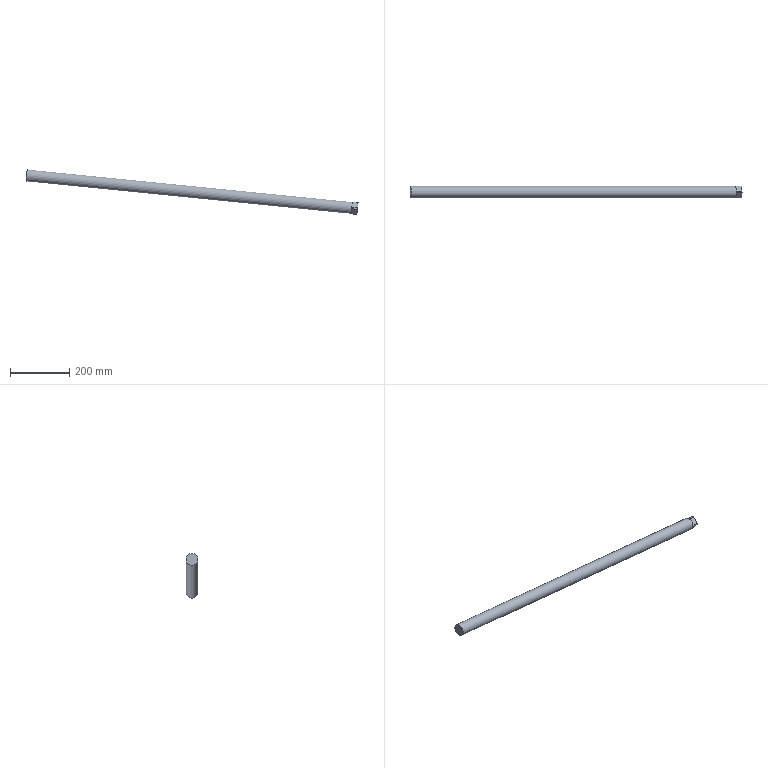Component | NX | ADJUSTTABLE_AXLE1 | 2 solids | 13 faces | box 1123.41 x 40 x 151.52 mm | volume 1408479 mm3 | plane 8 | other 4 | cylinder 1 | commonest cylinder face diameters 40 x1
STEP:
#1=CARTESIAN_POINT('',(0.,0.,0.));
#2=DIRECTION('',(0.,0.,1.));
#3=DIRECTION('',(1.,0.,0.));
#4=AXIS2_PLACEMENT_3D('',#1,#2,#3);
#5=CARTESIAN_POINT('',(1583.185,87.5,396.935));
#6=VERTEX_POINT('',#5);
#7=CARTESIAN_POINT('',(1583.185,67.5,396.935));
#8=DIRECTION('',(0.9951,0.,-0.09932));
#9=DIRECTION('',(0.,1.,0.));
#10=AXIS2_PLACEMENT_3D('',#7,#8,#9);
#11=CIRCLE('',#10,20.);
#12=CARTESIAN_POINT('',(1583.185,67.5,396.935));
#13=DIRECTION('',(-0.9951,0.,0.09932));
#14=DIRECTION('',(0.09932,0.,0.9951));
#15=AXIS2_PLACEMENT_3D('',#12,#13,#14);
#16=CYLINDRICAL_SURFACE('',#15,20.);
#17=CARTESIAN_POINT('',(7.854,0.));
#18=DIRECTION('',(-1.,0.));
#19=VECTOR('',#18,1.);
#20=LINE('',#17,#19);
#21=(GEOMETRIC_REPRESENTATION_CONTEXT(2)PARAMETRIC_REPRESENTATION_CONTEXT()REPRESENTATION_CONTEXT('',''));
#22=DEFINITIONAL_REPRESENTATION('',(#20),#21);
#23=PCURVE('',#16,#22);
#24=CARTESIAN_POINT('',(1583.185,67.5,396.935));
#25=DIRECTION('',(0.9951,0.,-0.09932));
#26=DIRECTION('',(-0.09932,0.,-0.9951));
#27=AXIS2_PLACEMENT_3D('',#24,#25,#26);
#28=PLANE('',#27);
#29=CARTESIAN_POINT('',(0.,0.));
#30=DIRECTION('',(0.,1.));
#31=AXIS2_PLACEMENT_2D('',#29,#30);
#32=CIRCLE('',#31,20.);
#33=(GEOMETRIC_REPRESENTATION_CONTEXT(2)PARAMETRIC_REPRESENTATION_CONTEXT()REPRESENTATION_CONTEXT('',''));
#34=DEFINITIONAL_REPRESENTATION('',(#32),#33);
#35=PCURVE('',#28,#34);
#36=SURFACE_CURVE('',#11,(#23,#35),.PCURVE_S1.);
#37=EDGE_CURVE('',#6,#6,#36,.T.);
#38=ORIENTED_EDGE('',*,*,#37,.F.);
#39=CARTESIAN_POINT('',(483.649,87.5,506.684));
#40=VERTEX_POINT('',#39);
#41=CARTESIAN_POINT('',(1583.185,87.5,396.935));
#42=CARTESIAN_POINT('',(483.649,87.5,506.684));
#43=B_SPLINE_CURVE_WITH_KNOTS('',1,(#41,#42),.UNSPECIFIED.,.F.,.F.,(2,2),(0.,1105.),.PIECEWISE_BEZIER_KNOTS.);
#44=CARTESIAN_POINT('',(7.854,0.));
#45=DIRECTION('',(0.,1.));
#46=VECTOR('',#45,1.);
#47=LINE('',#44,#46);
#48=(GEOMETRIC_REPRESENTATION_CONTEXT(2)PARAMETRIC_REPRESENTATION_CONTEXT()REPRESENTATION_CONTEXT('',''));
#49=DEFINITIONAL_REPRESENTATION('',(#47),#48);
#50=PCURVE('',#16,#49);
#51=CARTESIAN_POINT('',(1.571,0.));
#52=DIRECTION('',(0.,1.));
#53=VECTOR('',#52,1.);
#54=LINE('',#51,#53);
#55=(GEOMETRIC_REPRESENTATION_CONTEXT(2)PARAMETRIC_REPRESENTATION_CONTEXT()REPRESENTATION_CONTEXT('',''));
#56=DEFINITIONAL_REPRESENTATION('',(#54),#55);
#57=PCURVE('',#16,#56);
#58=SEAM_CURVE('',#43,(#50,#57),.PCURVE_S1.);
#59=EDGE_CURVE('',#6,#40,#58,.T.);
#60=ORIENTED_EDGE('',*,*,#59,.T.);
#61=CARTESIAN_POINT('',(483.649,67.5,506.684));
#62=DIRECTION('',(0.9951,0.,-0.09932));
#63=DIRECTION('',(0.,1.,0.));
#64=AXIS2_PLACEMENT_3D('',#61,#62,#63);
#65=CIRCLE('',#64,20.);
#66=CARTESIAN_POINT('',(7.854,1105.));
#67=DIRECTION('',(-1.,0.));
#68=VECTOR('',#67,1.);
#69=LINE('',#66,#68);
#70=(GEOMETRIC_REPRESENTATION_CONTEXT(2)PARAMETRIC_REPRESENTATION_CONTEXT()REPRESENTATION_CONTEXT('',''));
#71=DEFINITIONAL_REPRESENTATION('',(#69),#70);
#72=PCURVE('',#16,#71);
#73=CARTESIAN_POINT('',(483.649,67.5,506.684));
#74=DIRECTION('',(0.9951,0.,-0.09932));
#75=DIRECTION('',(-0.09932,0.,-0.9951));
#76=AXIS2_PLACEMENT_3D('',#73,#74,#75);
#77=PLANE('',#76);
#78=CARTESIAN_POINT('',(0.,0.));
#79=DIRECTION('',(0.,1.));
#80=AXIS2_PLACEMENT_2D('',#78,#79);
#81=CIRCLE('',#80,20.);
#82=(GEOMETRIC_REPRESENTATION_CONTEXT(2)PARAMETRIC_REPRESENTATION_CONTEXT()REPRESENTATION_CONTEXT('',''));
#83=DEFINITIONAL_REPRESENTATION('',(#81),#82);
#84=PCURVE('',#77,#83);
#85=SURFACE_CURVE('',#65,(#72,#84),.PCURVE_S1.);
#86=EDGE_CURVE('',#40,#40,#85,.T.);
#87=ORIENTED_EDGE('',*,*,#86,.T.);
#88=ORIENTED_EDGE('',*,*,#59,.F.);
#89=EDGE_LOOP('',(#38,#60,#87,#88));
#90=FACE_BOUND('',#89,.T.);
#91=ADVANCED_FACE('',(#90),#16,.T.);
#92=ORIENTED_EDGE('',*,*,#37,.T.);
#93=EDGE_LOOP('',(#92));
#94=FACE_BOUND('',#93,.T.);
#95=ADVANCED_FACE('',(#94),#28,.T.);
#96=ORIENTED_EDGE('',*,*,#86,.F.);
#97=EDGE_LOOP('',(#96));
#98=FACE_BOUND('',#97,.T.);
#99=ADVANCED_FACE('',(#98),#77,.F.);
#100=CLOSED_SHELL('',(#91,#95,#99));
#101=MANIFOLD_SOLID_BREP('',#100);
#102=(LENGTH_UNIT()NAMED_UNIT(*)SI_UNIT(.MILLI.,.METRE.));
#103=UNCERTAINTY_MEASURE_WITH_UNIT(LENGTH_MEASURE(0.00001),#102,'','');
#104=(NAMED_UNIT(*)PLANE_ANGLE_UNIT()SI_UNIT($,.RADIAN.));
#105=(NAMED_UNIT(*)SI_UNIT($,.STERADIAN.)SOLID_ANGLE_UNIT());
#106=(GEOMETRIC_REPRESENTATION_CONTEXT(3)GLOBAL_UNCERTAINTY_ASSIGNED_CONTEXT((#103))GLOBAL_UNIT_ASSIGNED_CONTEXT((#102,#104,#105))REPRESENTATION_CONTEXT('',''));
#107=ADVANCED_BREP_SHAPE_REPRESENTATION('',(#4,#101),#106);
#108=CARTESIAN_POINT('',(0.,0.,0.));
#109=DIRECTION('',(0.,0.,1.));
#110=DIRECTION('',(1.,0.,0.));
#111=AXIS2_PLACEMENT_3D('',#108,#109,#110);
#112=CARTESIAN_POINT('',(0.,0.,0.));
#113=DIRECTION('',(0.,0.,1.));
#114=DIRECTION('',(1.,0.,0.));
#115=AXIS2_PLACEMENT_3D('',#112,#113,#114);
#116=(LENGTH_UNIT()NAMED_UNIT(*)SI_UNIT(.MILLI.,.METRE.));
#117=UNCERTAINTY_MEASURE_WITH_UNIT(LENGTH_MEASURE(0.000001),#116,'','');
#118=(NAMED_UNIT(*)PLANE_ANGLE_UNIT()SI_UNIT($,.RADIAN.));
#119=(NAMED_UNIT(*)SI_UNIT($,.STERADIAN.)SOLID_ANGLE_UNIT());
#120=(GEOMETRIC_REPRESENTATION_CONTEXT(3)GLOBAL_UNCERTAINTY_ASSIGNED_CONTEXT((#117))GLOBAL_UNIT_ASSIGNED_CONTEXT((#116,#118,#119))REPRESENTATION_CONTEXT('',''));
#121=SHAPE_REPRESENTATION('',(#4,#111,#115),#120);
#122=ITEM_DEFINED_TRANSFORMATION('','',#4,#111);
#123=(REPRESENTATION_RELATIONSHIP('','',#107,#121)REPRESENTATION_RELATIONSHIP_WITH_TRANSFORMATION(#122)SHAPE_REPRESENTATION_RELATIONSHIP());
#124=CARTESIAN_POINT('',(1603.368,47.704,397.767));
#125=VERTEX_POINT('',#124);
#126=CARTESIAN_POINT('',(1583.467,47.704,399.753));
#127=VERTEX_POINT('',#126);
#128=CARTESIAN_POINT('',(1603.368,47.704,397.767));
#129=DIRECTION('',(-0.9951,0.,0.09932));
#130=VECTOR('',#129,1.);
#131=LINE('',#128,#130);
#132=CARTESIAN_POINT('',(1603.086,67.5,394.949));
#133=DIRECTION('',(0.9951,0.,-0.09932));
#134=DIRECTION('',(0.,1.,0.));
#135=AXIS2_PLACEMENT_3D('',#132,#133,#134);
#136=ELLIPSE('',#135,19.997,19.98);
#137=DIRECTION('',(-0.9951,0.,0.09932));
#138=VECTOR('',#137,1.);
#139=SURFACE_OF_LINEAR_EXTRUSION('',#136,#138);
#140=CARTESIAN_POINT('',(2.999,-0.));
#141=DIRECTION('',(0.,1.));
#142=VECTOR('',#141,1.);
#143=LINE('',#140,#142);
#144=(GEOMETRIC_REPRESENTATION_CONTEXT(2)PARAMETRIC_REPRESENTATION_CONTEXT()REPRESENTATION_CONTEXT('',''));
#145=DEFINITIONAL_REPRESENTATION('',(#143),#144);
#146=PCURVE('',#139,#145);
#147=CARTESIAN_POINT('',(1605.05,64.648,414.627));
#148=DIRECTION('',(-0.07023,0.7071,-0.7036));
#149=DIRECTION('',(0.07023,0.7071,0.7036));
#150=AXIS2_PLACEMENT_3D('',#147,#148,#149);
#151=PLANE('',#150);
#152=CARTESIAN_POINT('',(-23.962,0.));
#153=DIRECTION('',(0.,-1.));
#154=VECTOR('',#153,1.);
#155=LINE('',#152,#154);
#156=(GEOMETRIC_REPRESENTATION_CONTEXT(2)PARAMETRIC_REPRESENTATION_CONTEXT()REPRESENTATION_CONTEXT('',''));
#157=DEFINITIONAL_REPRESENTATION('',(#155),#156);
#158=PCURVE('',#151,#157);
#159=SURFACE_CURVE('',#131,(#146,#158),.PCURVE_S1.);
#160=EDGE_CURVE('',#125,#127,#159,.T.);
#161=ORIENTED_EDGE('',*,*,#160,.F.);
#162=CARTESIAN_POINT('',(1602.805,47.704,392.131));
#163=VERTEX_POINT('',#162);
#164=CARTESIAN_POINT('',(1603.086,67.5,394.949));
#165=DIRECTION('',(0.9951,0.,-0.09932));
#166=DIRECTION('',(0.,1.,0.));
#167=AXIS2_PLACEMENT_3D('',#164,#165,#166);
#168=ELLIPSE('',#167,19.997,19.98);
#169=CARTESIAN_POINT('',(0.,0.));
#170=DIRECTION('',(1.,0.));
#171=VECTOR('',#170,1.);
#172=LINE('',#169,#171);
#173=(GEOMETRIC_REPRESENTATION_CONTEXT(2)PARAMETRIC_REPRESENTATION_CONTEXT()REPRESENTATION_CONTEXT('',''));
#174=DEFINITIONAL_REPRESENTATION('',(#172),#173);
#175=PCURVE('',#139,#174);
#176=CARTESIAN_POINT('',(1603.086,67.5,394.949));
#177=DIRECTION('',(0.9951,0.,-0.09932));
#178=DIRECTION('',(-0.09932,0.,-0.9951));
#179=AXIS2_PLACEMENT_3D('',#176,#177,#178);
#180=PLANE('',#179);
#181=CARTESIAN_POINT('',(0.,0.));
#182=DIRECTION('',(0.,1.));
#183=AXIS2_PLACEMENT_2D('',#181,#182);
#184=ELLIPSE('',#183,19.997,19.98);
#185=(GEOMETRIC_REPRESENTATION_CONTEXT(2)PARAMETRIC_REPRESENTATION_CONTEXT()REPRESENTATION_CONTEXT('',''));
#186=DEFINITIONAL_REPRESENTATION('',(#184),#185);
#187=PCURVE('',#180,#186);
#188=SURFACE_CURVE('',#168,(#175,#187),.PCURVE_S1.);
#189=EDGE_CURVE('',#125,#163,#188,.T.);
#190=ORIENTED_EDGE('',*,*,#189,.T.);
#191=CARTESIAN_POINT('',(1582.904,47.704,394.118));
#192=VERTEX_POINT('',#191);
#193=CARTESIAN_POINT('',(1602.805,47.704,392.131));
#194=DIRECTION('',(-0.9951,0.,0.09932));
#195=VECTOR('',#194,1.);
#196=LINE('',#193,#195);
#197=CARTESIAN_POINT('',(3.284,-0.));
#198=DIRECTION('',(0.,1.));
#199=VECTOR('',#198,1.);
#200=LINE('',#197,#199);
#201=(GEOMETRIC_REPRESENTATION_CONTEXT(2)PARAMETRIC_REPRESENTATION_CONTEXT()REPRESENTATION_CONTEXT('',''));
#202=DEFINITIONAL_REPRESENTATION('',(#200),#201);
#203=PCURVE('',#139,#202);
#204=CARTESIAN_POINT('',(1602.805,47.704,392.131));
#205=DIRECTION('',(0.07023,0.7071,0.7036));
#206=DIRECTION('',(0.07023,-0.7071,0.7036));
#207=AXIS2_PLACEMENT_3D('',#204,#205,#206);
#208=PLANE('',#207);
#209=CARTESIAN_POINT('',(-0.,-0.));
#210=DIRECTION('',(0.,-1.));
#211=VECTOR('',#210,1.);
#212=LINE('',#209,#211);
#213=(GEOMETRIC_REPRESENTATION_CONTEXT(2)PARAMETRIC_REPRESENTATION_CONTEXT()REPRESENTATION_CONTEXT('',''));
#214=DEFINITIONAL_REPRESENTATION('',(#212),#213);
#215=PCURVE('',#208,#214);
#216=SURFACE_CURVE('',#196,(#203,#215),.PCURVE_S1.);
#217=EDGE_CURVE('',#163,#192,#216,.T.);
#218=ORIENTED_EDGE('',*,*,#217,.T.);
#219=CARTESIAN_POINT('',(1583.185,67.5,396.935));
#220=DIRECTION('',(0.9951,0.,-0.09932));
#221=DIRECTION('',(0.,1.,0.));
#222=AXIS2_PLACEMENT_3D('',#219,#220,#221);
#223=ELLIPSE('',#222,19.997,19.98);
#224=CARTESIAN_POINT('',(-0.,20.));
#225=DIRECTION('',(1.,-0.));
#226=VECTOR('',#225,1.);
#227=LINE('',#224,#226);
#228=(GEOMETRIC_REPRESENTATION_CONTEXT(2)PARAMETRIC_REPRESENTATION_CONTEXT()REPRESENTATION_CONTEXT('',''));
#229=DEFINITIONAL_REPRESENTATION('',(#227),#228);
#230=PCURVE('',#139,#229);
#231=CARTESIAN_POINT('',(1583.185,67.5,396.935));
#232=DIRECTION('',(0.9951,0.,-0.09932));
#233=DIRECTION('',(-0.09932,0.,-0.9951));
#234=AXIS2_PLACEMENT_3D('',#231,#232,#233);
#235=PLANE('',#234);
#236=CARTESIAN_POINT('',(0.,0.));
#237=DIRECTION('',(0.,1.));
#238=AXIS2_PLACEMENT_2D('',#236,#237);
#239=ELLIPSE('',#238,19.997,19.98);
#240=(GEOMETRIC_REPRESENTATION_CONTEXT(2)PARAMETRIC_REPRESENTATION_CONTEXT()REPRESENTATION_CONTEXT('',''));
#241=DEFINITIONAL_REPRESENTATION('',(#239),#240);
#242=PCURVE('',#235,#241);
#243=SURFACE_CURVE('',#223,(#230,#242),.PCURVE_S1.);
#244=EDGE_CURVE('',#127,#192,#243,.T.);
#245=ORIENTED_EDGE('',*,*,#244,.F.);
#246=EDGE_LOOP('',(#161,#190,#218,#245));
#247=FACE_BOUND('',#246,.F.);
#248=ADVANCED_FACE('',(#247),#139,.F.);
#249=CARTESIAN_POINT('',(1581.221,64.648,377.258));
#250=VERTEX_POINT('',#249);
#251=CARTESIAN_POINT('',(1582.904,47.704,394.118));
#252=DIRECTION('',(-0.07023,0.7071,-0.7036));
#253=VECTOR('',#252,1.);
#254=LINE('',#251,#253);
#255=CARTESIAN_POINT('',(-0.,-20.));
#256=DIRECTION('',(-1.,-0.));
#257=VECTOR('',#256,1.);
#258=LINE('',#255,#257);
#259=(GEOMETRIC_REPRESENTATION_CONTEXT(2)PARAMETRIC_REPRESENTATION_CONTEXT()REPRESENTATION_CONTEXT('',''));
#260=DEFINITIONAL_REPRESENTATION('',(#258),#259);
#261=PCURVE('',#208,#260);
#262=CARTESIAN_POINT('',(2.832,-19.796));
#263=DIRECTION('',(0.7071,0.7071));
#264=VECTOR('',#263,1.);
#265=LINE('',#262,#264);
#266=(GEOMETRIC_REPRESENTATION_CONTEXT(2)PARAMETRIC_REPRESENTATION_CONTEXT()REPRESENTATION_CONTEXT('',''));
#267=DEFINITIONAL_REPRESENTATION('',(#265),#266);
#268=PCURVE('',#235,#267);
#269=SURFACE_CURVE('',#254,(#261,#268),.PCURVE_S1.);
#270=EDGE_CURVE('',#192,#250,#269,.T.);
#271=ORIENTED_EDGE('',*,*,#270,.T.);
#272=CARTESIAN_POINT('',(1601.122,64.648,375.271));
#273=VERTEX_POINT('',#272);
#274=CARTESIAN_POINT('',(1601.122,64.648,375.271));
#275=DIRECTION('',(-0.9951,0.,0.09932));
#276=VECTOR('',#275,1.);
#277=LINE('',#274,#276);
#278=CARTESIAN_POINT('',(-23.962,-0.));
#279=DIRECTION('',(0.,-1.));
#280=VECTOR('',#279,1.);
#281=LINE('',#278,#280);
#282=(GEOMETRIC_REPRESENTATION_CONTEXT(2)PARAMETRIC_REPRESENTATION_CONTEXT()REPRESENTATION_CONTEXT('',''));
#283=DEFINITIONAL_REPRESENTATION('',(#281),#282);
#284=PCURVE('',#208,#283);
#285=CARTESIAN_POINT('',(1603.086,67.5,394.949));
#286=DIRECTION('',(0.9951,0.,-0.09932));
#287=DIRECTION('',(0.,1.,0.));
#288=AXIS2_PLACEMENT_3D('',#285,#286,#287);
#289=ELLIPSE('',#288,19.997,19.98);
#290=DIRECTION('',(-0.9951,0.,0.09932));
#291=VECTOR('',#290,1.);
#292=SURFACE_OF_LINEAR_EXTRUSION('',#289,#291);
#293=CARTESIAN_POINT('',(4.569,-0.));
#294=DIRECTION('',(0.,1.));
#295=VECTOR('',#294,1.);
#296=LINE('',#293,#295);
#297=(GEOMETRIC_REPRESENTATION_CONTEXT(2)PARAMETRIC_REPRESENTATION_CONTEXT()REPRESENTATION_CONTEXT('',''));
#298=DEFINITIONAL_REPRESENTATION('',(#296),#297);
#299=PCURVE('',#292,#298);
#300=SURFACE_CURVE('',#277,(#284,#299),.PCURVE_S1.);
#301=EDGE_CURVE('',#273,#250,#300,.T.);
#302=ORIENTED_EDGE('',*,*,#301,.F.);
#303=CARTESIAN_POINT('',(1602.805,47.704,392.131));
#304=DIRECTION('',(-0.07023,0.7071,-0.7036));
#305=VECTOR('',#304,1.);
#306=LINE('',#303,#305);
#307=CARTESIAN_POINT('',(0.,0.));
#308=DIRECTION('',(-1.,-0.));
#309=VECTOR('',#308,1.);
#310=LINE('',#307,#309);
#311=(GEOMETRIC_REPRESENTATION_CONTEXT(2)PARAMETRIC_REPRESENTATION_CONTEXT()REPRESENTATION_CONTEXT('',''));
#312=DEFINITIONAL_REPRESENTATION('',(#310),#311);
#313=PCURVE('',#208,#312);
#314=CARTESIAN_POINT('',(2.832,-19.796));
#315=DIRECTION('',(0.7071,0.7071));
#316=VECTOR('',#315,1.);
#317=LINE('',#314,#316);
#318=(GEOMETRIC_REPRESENTATION_CONTEXT(2)PARAMETRIC_REPRESENTATION_CONTEXT()REPRESENTATION_CONTEXT('',''));
#319=DEFINITIONAL_REPRESENTATION('',(#317),#318);
#320=PCURVE('',#180,#319);
#321=SURFACE_CURVE('',#306,(#313,#320),.PCURVE_S1.);
#322=EDGE_CURVE('',#163,#273,#321,.T.);
#323=ORIENTED_EDGE('',*,*,#322,.F.);
#324=ORIENTED_EDGE('',*,*,#217,.T.);
#325=EDGE_LOOP('',(#271,#302,#323,#324));
#326=FACE_BOUND('',#325,.T.);
#327=ADVANCED_FACE('',(#326),#208,.F.);
#328=ORIENTED_EDGE('',*,*,#301,.F.);
#329=CARTESIAN_POINT('',(1601.122,70.352,375.271));
#330=VERTEX_POINT('',#329);
#331=CARTESIAN_POINT('',(1603.086,67.5,394.949));
#332=DIRECTION('',(0.9951,0.,-0.09932));
#333=DIRECTION('',(0.,1.,0.));
#334=AXIS2_PLACEMENT_3D('',#331,#332,#333);
#335=ELLIPSE('',#334,19.997,19.98);
#336=CARTESIAN_POINT('',(0.,0.));
#337=DIRECTION('',(1.,0.));
#338=VECTOR('',#337,1.);
#339=LINE('',#336,#338);
#340=(GEOMETRIC_REPRESENTATION_CONTEXT(2)PARAMETRIC_REPRESENTATION_CONTEXT()REPRESENTATION_CONTEXT('',''));
#341=DEFINITIONAL_REPRESENTATION('',(#339),#340);
#342=PCURVE('',#292,#341);
#343=CARTESIAN_POINT('',(0.,0.));
#344=DIRECTION('',(0.,1.));
#345=AXIS2_PLACEMENT_2D('',#343,#344);
#346=ELLIPSE('',#345,19.997,19.98);
#347=(GEOMETRIC_REPRESENTATION_CONTEXT(2)PARAMETRIC_REPRESENTATION_CONTEXT()REPRESENTATION_CONTEXT('',''));
#348=DEFINITIONAL_REPRESENTATION('',(#346),#347);
#349=PCURVE('',#180,#348);
#350=SURFACE_CURVE('',#335,(#342,#349),.PCURVE_S1.);
#351=EDGE_CURVE('',#273,#330,#350,.T.);
#352=ORIENTED_EDGE('',*,*,#351,.T.);
#353=CARTESIAN_POINT('',(1581.221,70.352,377.258));
#354=VERTEX_POINT('',#353);
#355=CARTESIAN_POINT('',(1601.122,70.352,375.271));
#356=DIRECTION('',(-0.9951,0.,0.09932));
#357=VECTOR('',#356,1.);
#358=LINE('',#355,#357);
#359=CARTESIAN_POINT('',(4.855,-0.));
#360=DIRECTION('',(-0.,1.));
#361=VECTOR('',#360,1.);
#362=LINE('',#359,#361);
#363=(GEOMETRIC_REPRESENTATION_CONTEXT(2)PARAMETRIC_REPRESENTATION_CONTEXT()REPRESENTATION_CONTEXT('',''));
#364=DEFINITIONAL_REPRESENTATION('',(#362),#363);
#365=PCURVE('',#292,#364);
#366=CARTESIAN_POINT('',(1601.122,70.352,375.271));
#367=DIRECTION('',(0.07023,-0.7071,0.7036));
#368=DIRECTION('',(-0.07023,-0.7071,-0.7036));
#369=AXIS2_PLACEMENT_3D('',#366,#367,#368);
#370=PLANE('',#369);
#371=CARTESIAN_POINT('',(0.,0.));
#372=DIRECTION('',(0.,-1.));
#373=VECTOR('',#372,1.);
#374=LINE('',#371,#373);
#375=(GEOMETRIC_REPRESENTATION_CONTEXT(2)PARAMETRIC_REPRESENTATION_CONTEXT()REPRESENTATION_CONTEXT('',''));
#376=DEFINITIONAL_REPRESENTATION('',(#374),#375);
#377=PCURVE('',#370,#376);
#378=SURFACE_CURVE('',#358,(#365,#377),.PCURVE_S1.);
#379=EDGE_CURVE('',#330,#354,#378,.T.);
#380=ORIENTED_EDGE('',*,*,#379,.T.);
#381=CARTESIAN_POINT('',(1583.185,67.5,396.935));
#382=DIRECTION('',(0.9951,0.,-0.09932));
#383=DIRECTION('',(0.,1.,0.));
#384=AXIS2_PLACEMENT_3D('',#381,#382,#383);
#385=ELLIPSE('',#384,19.997,19.98);
#386=CARTESIAN_POINT('',(-0.,20.));
#387=DIRECTION('',(1.,0.));
#388=VECTOR('',#387,1.);
#389=LINE('',#386,#388);
#390=(GEOMETRIC_REPRESENTATION_CONTEXT(2)PARAMETRIC_REPRESENTATION_CONTEXT()REPRESENTATION_CONTEXT('',''));
#391=DEFINITIONAL_REPRESENTATION('',(#389),#390);
#392=PCURVE('',#292,#391);
#393=CARTESIAN_POINT('',(0.,0.));
#394=DIRECTION('',(0.,1.));
#395=AXIS2_PLACEMENT_2D('',#393,#394);
#396=ELLIPSE('',#395,19.997,19.98);
#397=(GEOMETRIC_REPRESENTATION_CONTEXT(2)PARAMETRIC_REPRESENTATION_CONTEXT()REPRESENTATION_CONTEXT('',''));
#398=DEFINITIONAL_REPRESENTATION('',(#396),#397);
#399=PCURVE('',#235,#398);
#400=SURFACE_CURVE('',#385,(#392,#399),.PCURVE_S1.);
#401=EDGE_CURVE('',#250,#354,#400,.T.);
#402=ORIENTED_EDGE('',*,*,#401,.F.);
#403=EDGE_LOOP('',(#328,#352,#380,#402));
#404=FACE_BOUND('',#403,.F.);
#405=ADVANCED_FACE('',(#404),#292,.F.);
#406=CARTESIAN_POINT('',(1582.904,87.296,394.118));
#407=VERTEX_POINT('',#406);
#408=CARTESIAN_POINT('',(1581.221,70.352,377.258));
#409=DIRECTION('',(0.07023,0.7071,0.7036));
#410=VECTOR('',#409,1.);
#411=LINE('',#408,#410);
#412=CARTESIAN_POINT('',(-0.,-20.));
#413=DIRECTION('',(-1.,-0.));
#414=VECTOR('',#413,1.);
#415=LINE('',#412,#414);
#416=(GEOMETRIC_REPRESENTATION_CONTEXT(2)PARAMETRIC_REPRESENTATION_CONTEXT()REPRESENTATION_CONTEXT('',''));
#417=DEFINITIONAL_REPRESENTATION('',(#415),#416);
#418=PCURVE('',#370,#417);
#419=CARTESIAN_POINT('',(19.775,2.852));
#420=DIRECTION('',(-0.7071,0.7071));
#421=VECTOR('',#420,1.);
#422=LINE('',#419,#421);
#423=(GEOMETRIC_REPRESENTATION_CONTEXT(2)PARAMETRIC_REPRESENTATION_CONTEXT()REPRESENTATION_CONTEXT('',''));
#424=DEFINITIONAL_REPRESENTATION('',(#422),#423);
#425=PCURVE('',#235,#424);
#426=SURFACE_CURVE('',#411,(#418,#425),.PCURVE_S1.);
#427=EDGE_CURVE('',#354,#407,#426,.T.);
#428=ORIENTED_EDGE('',*,*,#427,.T.);
#429=CARTESIAN_POINT('',(1602.805,87.296,392.131));
#430=VERTEX_POINT('',#429);
#431=CARTESIAN_POINT('',(1602.805,87.296,392.131));
#432=DIRECTION('',(-0.9951,0.,0.09932));
#433=VECTOR('',#432,1.);
#434=LINE('',#431,#433);
#435=CARTESIAN_POINT('',(-23.962,0.));
#436=DIRECTION('',(0.,-1.));
#437=VECTOR('',#436,1.);
#438=LINE('',#435,#437);
#439=(GEOMETRIC_REPRESENTATION_CONTEXT(2)PARAMETRIC_REPRESENTATION_CONTEXT()REPRESENTATION_CONTEXT('',''));
#440=DEFINITIONAL_REPRESENTATION('',(#438),#439);
#441=PCURVE('',#370,#440);
#442=CARTESIAN_POINT('',(1603.086,67.5,394.949));
#443=DIRECTION('',(0.9951,0.,-0.09932));
#444=DIRECTION('',(0.,1.,0.));
#445=AXIS2_PLACEMENT_3D('',#442,#443,#444);
#446=ELLIPSE('',#445,19.997,19.98);
#447=DIRECTION('',(-0.9951,0.,0.09932));
#448=VECTOR('',#447,1.);
#449=SURFACE_OF_LINEAR_EXTRUSION('',#446,#448);
#450=CARTESIAN_POINT('',(-0.1422,-0.));
#451=DIRECTION('',(0.,1.));
#452=VECTOR('',#451,1.);
#453=LINE('',#450,#452);
#454=(GEOMETRIC_REPRESENTATION_CONTEXT(2)PARAMETRIC_REPRESENTATION_CONTEXT()REPRESENTATION_CONTEXT('',''));
#455=DEFINITIONAL_REPRESENTATION('',(#453),#454);
#456=PCURVE('',#449,#455);
#457=SURFACE_CURVE('',#434,(#441,#456),.PCURVE_S1.);
#458=EDGE_CURVE('',#430,#407,#457,.T.);
#459=ORIENTED_EDGE('',*,*,#458,.F.);
#460=CARTESIAN_POINT('',(1601.122,70.352,375.271));
#461=DIRECTION('',(0.07023,0.7071,0.7036));
#462=VECTOR('',#461,1.);
#463=LINE('',#460,#462);
#464=CARTESIAN_POINT('',(0.,0.));
#465=DIRECTION('',(-1.,-0.));
#466=VECTOR('',#465,1.);
#467=LINE('',#464,#466);
#468=(GEOMETRIC_REPRESENTATION_CONTEXT(2)PARAMETRIC_REPRESENTATION_CONTEXT()REPRESENTATION_CONTEXT('',''));
#469=DEFINITIONAL_REPRESENTATION('',(#467),#468);
#470=PCURVE('',#370,#469);
#471=CARTESIAN_POINT('',(19.775,2.852));
#472=DIRECTION('',(-0.7071,0.7071));
#473=VECTOR('',#472,1.);
#474=LINE('',#471,#473);
#475=(GEOMETRIC_REPRESENTATION_CONTEXT(2)PARAMETRIC_REPRESENTATION_CONTEXT()REPRESENTATION_CONTEXT('',''));
#476=DEFINITIONAL_REPRESENTATION('',(#474),#475);
#477=PCURVE('',#180,#476);
#478=SURFACE_CURVE('',#463,(#470,#477),.PCURVE_S1.);
#479=EDGE_CURVE('',#330,#430,#478,.T.);
#480=ORIENTED_EDGE('',*,*,#479,.F.);
#481=ORIENTED_EDGE('',*,*,#379,.T.);
#482=EDGE_LOOP('',(#428,#459,#480,#481));
#483=FACE_BOUND('',#482,.T.);
#484=ADVANCED_FACE('',(#483),#370,.F.);
#485=ORIENTED_EDGE('',*,*,#458,.F.);
#486=CARTESIAN_POINT('',(1603.368,87.296,397.767));
#487=VERTEX_POINT('',#486);
#488=CARTESIAN_POINT('',(1603.086,67.5,394.949));
#489=DIRECTION('',(0.9951,0.,-0.09932));
#490=DIRECTION('',(0.,1.,0.));
#491=AXIS2_PLACEMENT_3D('',#488,#489,#490);
#492=ELLIPSE('',#491,19.997,19.98);
#493=CARTESIAN_POINT('',(-6.283,-0.));
#494=DIRECTION('',(1.,0.));
#495=VECTOR('',#494,1.);
#496=LINE('',#493,#495);
#497=(GEOMETRIC_REPRESENTATION_CONTEXT(2)PARAMETRIC_REPRESENTATION_CONTEXT()REPRESENTATION_CONTEXT('',''));
#498=DEFINITIONAL_REPRESENTATION('',(#496),#497);
#499=PCURVE('',#449,#498);
#500=CARTESIAN_POINT('',(0.,0.));
#501=DIRECTION('',(0.,1.));
#502=AXIS2_PLACEMENT_2D('',#500,#501);
#503=ELLIPSE('',#502,19.997,19.98);
#504=(GEOMETRIC_REPRESENTATION_CONTEXT(2)PARAMETRIC_REPRESENTATION_CONTEXT()REPRESENTATION_CONTEXT('',''));
#505=DEFINITIONAL_REPRESENTATION('',(#503),#504);
#506=PCURVE('',#180,#505);
#507=SURFACE_CURVE('',#492,(#499,#506),.PCURVE_S1.);
#508=EDGE_CURVE('',#430,#487,#507,.T.);
#509=ORIENTED_EDGE('',*,*,#508,.T.);
#510=CARTESIAN_POINT('',(1583.467,87.296,399.753));
#511=VERTEX_POINT('',#510);
#512=CARTESIAN_POINT('',(1603.368,87.296,397.767));
#513=DIRECTION('',(-0.9951,0.,0.09932));
#514=VECTOR('',#513,1.);
#515=LINE('',#512,#514);
#516=CARTESIAN_POINT('',(0.1422,-0.));
#517=DIRECTION('',(0.,1.));
#518=VECTOR('',#517,1.);
#519=LINE('',#516,#518);
#520=(GEOMETRIC_REPRESENTATION_CONTEXT(2)PARAMETRIC_REPRESENTATION_CONTEXT()REPRESENTATION_CONTEXT('',''));
#521=DEFINITIONAL_REPRESENTATION('',(#519),#520);
#522=PCURVE('',#449,#521);
#523=CARTESIAN_POINT('',(1603.368,87.296,397.767));
#524=DIRECTION('',(-0.07023,-0.7071,-0.7036));
#525=DIRECTION('',(-0.07023,0.7071,-0.7036));
#526=AXIS2_PLACEMENT_3D('',#523,#524,#525);
#527=PLANE('',#526);
#528=CARTESIAN_POINT('',(0.,0.));
#529=DIRECTION('',(0.,-1.));
#530=VECTOR('',#529,1.);
#531=LINE('',#528,#530);
#532=(GEOMETRIC_REPRESENTATION_CONTEXT(2)PARAMETRIC_REPRESENTATION_CONTEXT()REPRESENTATION_CONTEXT('',''));
#533=DEFINITIONAL_REPRESENTATION('',(#531),#532);
#534=PCURVE('',#527,#533);
#535=SURFACE_CURVE('',#515,(#522,#534),.PCURVE_S1.);
#536=EDGE_CURVE('',#487,#511,#535,.T.);
#537=ORIENTED_EDGE('',*,*,#536,.T.);
#538=CARTESIAN_POINT('',(1583.185,67.5,396.935));
#539=DIRECTION('',(0.9951,0.,-0.09932));
#540=DIRECTION('',(0.,1.,0.));
#541=AXIS2_PLACEMENT_3D('',#538,#539,#540);
#542=ELLIPSE('',#541,19.997,19.98);
#543=CARTESIAN_POINT('',(-6.283,20.));
#544=DIRECTION('',(1.,0.));
#545=VECTOR('',#544,1.);
#546=LINE('',#543,#545);
#547=(GEOMETRIC_REPRESENTATION_CONTEXT(2)PARAMETRIC_REPRESENTATION_CONTEXT()REPRESENTATION_CONTEXT('',''));
#548=DEFINITIONAL_REPRESENTATION('',(#546),#547);
#549=PCURVE('',#449,#548);
#550=CARTESIAN_POINT('',(0.,0.));
#551=DIRECTION('',(0.,1.));
#552=AXIS2_PLACEMENT_2D('',#550,#551);
#553=ELLIPSE('',#552,19.997,19.98);
#554=(GEOMETRIC_REPRESENTATION_CONTEXT(2)PARAMETRIC_REPRESENTATION_CONTEXT()REPRESENTATION_CONTEXT('',''));
#555=DEFINITIONAL_REPRESENTATION('',(#553),#554);
#556=PCURVE('',#235,#555);
#557=SURFACE_CURVE('',#542,(#549,#556),.PCURVE_S1.);
#558=EDGE_CURVE('',#407,#511,#557,.T.);
#559=ORIENTED_EDGE('',*,*,#558,.F.);
#560=EDGE_LOOP('',(#485,#509,#537,#559));
#561=FACE_BOUND('',#560,.F.);
#562=ADVANCED_FACE('',(#561),#449,.F.);
#563=CARTESIAN_POINT('',(1585.149,70.352,416.613));
#564=VERTEX_POINT('',#563);
#565=CARTESIAN_POINT('',(1583.467,87.296,399.753));
#566=DIRECTION('',(0.07023,-0.7071,0.7036));
#567=VECTOR('',#566,1.);
#568=LINE('',#565,#567);
#569=CARTESIAN_POINT('',(-0.,-20.));
#570=DIRECTION('',(-1.,-0.));
#571=VECTOR('',#570,1.);
#572=LINE('',#569,#571);
#573=(GEOMETRIC_REPRESENTATION_CONTEXT(2)PARAMETRIC_REPRESENTATION_CONTEXT()REPRESENTATION_CONTEXT('',''));
#574=DEFINITIONAL_REPRESENTATION('',(#572),#573);
#575=PCURVE('',#527,#574);
#576=CARTESIAN_POINT('',(-2.832,19.796));
#577=DIRECTION('',(-0.7071,-0.7071));
#578=VECTOR('',#577,1.);
#579=LINE('',#576,#578);
#580=(GEOMETRIC_REPRESENTATION_CONTEXT(2)PARAMETRIC_REPRESENTATION_CONTEXT()REPRESENTATION_CONTEXT('',''));
#581=DEFINITIONAL_REPRESENTATION('',(#579),#580);
#582=PCURVE('',#235,#581);
#583=SURFACE_CURVE('',#568,(#575,#582),.PCURVE_S1.);
#584=EDGE_CURVE('',#511,#564,#583,.T.);
#585=ORIENTED_EDGE('',*,*,#584,.T.);
#586=CARTESIAN_POINT('',(1605.05,70.352,414.627));
#587=VERTEX_POINT('',#586);
#588=CARTESIAN_POINT('',(1605.05,70.352,414.627));
#589=DIRECTION('',(-0.9951,0.,0.09932));
#590=VECTOR('',#589,1.);
#591=LINE('',#588,#590);
#592=CARTESIAN_POINT('',(-23.962,0.));
#593=DIRECTION('',(0.,-1.));
#594=VECTOR('',#593,1.);
#595=LINE('',#592,#594);
#596=(GEOMETRIC_REPRESENTATION_CONTEXT(2)PARAMETRIC_REPRESENTATION_CONTEXT()REPRESENTATION_CONTEXT('',''));
#597=DEFINITIONAL_REPRESENTATION('',(#595),#596);
#598=PCURVE('',#527,#597);
#599=CARTESIAN_POINT('',(1603.086,67.5,394.949));
#600=DIRECTION('',(0.9951,0.,-0.09932));
#601=DIRECTION('',(0.,1.,0.));
#602=AXIS2_PLACEMENT_3D('',#599,#600,#601);
#603=ELLIPSE('',#602,19.997,19.98);
#604=DIRECTION('',(-0.9951,0.,0.09932));
#605=VECTOR('',#604,1.);
#606=SURFACE_OF_LINEAR_EXTRUSION('',#603,#605);
#607=CARTESIAN_POINT('',(1.428,-0.));
#608=DIRECTION('',(0.,1.));
#609=VECTOR('',#608,1.);
#610=LINE('',#607,#609);
#611=(GEOMETRIC_REPRESENTATION_CONTEXT(2)PARAMETRIC_REPRESENTATION_CONTEXT()REPRESENTATION_CONTEXT('',''));
#612=DEFINITIONAL_REPRESENTATION('',(#610),#611);
#613=PCURVE('',#606,#612);
#614=SURFACE_CURVE('',#591,(#598,#613),.PCURVE_S1.);
#615=EDGE_CURVE('',#587,#564,#614,.T.);
#616=ORIENTED_EDGE('',*,*,#615,.F.);
#617=CARTESIAN_POINT('',(1603.368,87.296,397.767));
#618=DIRECTION('',(0.07023,-0.7071,0.7036));
#619=VECTOR('',#618,1.);
#620=LINE('',#617,#619);
#621=CARTESIAN_POINT('',(0.,0.));
#622=DIRECTION('',(-1.,-0.));
#623=VECTOR('',#622,1.);
#624=LINE('',#621,#623);
#625=(GEOMETRIC_REPRESENTATION_CONTEXT(2)PARAMETRIC_REPRESENTATION_CONTEXT()REPRESENTATION_CONTEXT('',''));
#626=DEFINITIONAL_REPRESENTATION('',(#624),#625);
#627=PCURVE('',#527,#626);
#628=CARTESIAN_POINT('',(-2.832,19.796));
#629=DIRECTION('',(-0.7071,-0.7071));
#630=VECTOR('',#629,1.);
#631=LINE('',#628,#630);
#632=(GEOMETRIC_REPRESENTATION_CONTEXT(2)PARAMETRIC_REPRESENTATION_CONTEXT()REPRESENTATION_CONTEXT('',''));
#633=DEFINITIONAL_REPRESENTATION('',(#631),#632);
#634=PCURVE('',#180,#633);
#635=SURFACE_CURVE('',#620,(#627,#634),.PCURVE_S1.);
#636=EDGE_CURVE('',#487,#587,#635,.T.);
#637=ORIENTED_EDGE('',*,*,#636,.F.);
#638=ORIENTED_EDGE('',*,*,#536,.T.);
#639=EDGE_LOOP('',(#585,#616,#637,#638));
#640=FACE_BOUND('',#639,.T.);
#641=ADVANCED_FACE('',(#640),#527,.F.);
#642=ORIENTED_EDGE('',*,*,#615,.F.);
#643=CARTESIAN_POINT('',(1605.05,64.648,414.627));
#644=VERTEX_POINT('',#643);
#645=CARTESIAN_POINT('',(1603.086,67.5,394.949));
#646=DIRECTION('',(0.9951,0.,-0.09932));
#647=DIRECTION('',(0.,1.,0.));
#648=AXIS2_PLACEMENT_3D('',#645,#646,#647);
#649=ELLIPSE('',#648,19.997,19.98);
#650=CARTESIAN_POINT('',(0.,-0.));
#651=DIRECTION('',(1.,0.));
#652=VECTOR('',#651,1.);
#653=LINE('',#650,#652);
#654=(GEOMETRIC_REPRESENTATION_CONTEXT(2)PARAMETRIC_REPRESENTATION_CONTEXT()REPRESENTATION_CONTEXT('',''));
#655=DEFINITIONAL_REPRESENTATION('',(#653),#654);
#656=PCURVE('',#606,#655);
#657=CARTESIAN_POINT('',(0.,0.));
#658=DIRECTION('',(0.,1.));
#659=AXIS2_PLACEMENT_2D('',#657,#658);
#660=ELLIPSE('',#659,19.997,19.98);
#661=(GEOMETRIC_REPRESENTATION_CONTEXT(2)PARAMETRIC_REPRESENTATION_CONTEXT()REPRESENTATION_CONTEXT('',''));
#662=DEFINITIONAL_REPRESENTATION('',(#660),#661);
#663=PCURVE('',#180,#662);
#664=SURFACE_CURVE('',#649,(#656,#663),.PCURVE_S1.);
#665=EDGE_CURVE('',#587,#644,#664,.T.);
#666=ORIENTED_EDGE('',*,*,#665,.T.);
#667=CARTESIAN_POINT('',(1585.149,64.648,416.613));
#668=VERTEX_POINT('',#667);
#669=CARTESIAN_POINT('',(1605.05,64.648,414.627));
#670=DIRECTION('',(-0.9951,0.,0.09932));
#671=VECTOR('',#670,1.);
#672=LINE('',#669,#671);
#673=CARTESIAN_POINT('',(1.714,-0.));
#674=DIRECTION('',(0.,1.));
#675=VECTOR('',#674,1.);
#676=LINE('',#673,#675);
#677=(GEOMETRIC_REPRESENTATION_CONTEXT(2)PARAMETRIC_REPRESENTATION_CONTEXT()REPRESENTATION_CONTEXT('',''));
#678=DEFINITIONAL_REPRESENTATION('',(#676),#677);
#679=PCURVE('',#606,#678);
#680=CARTESIAN_POINT('',(0.,0.));
#681=DIRECTION('',(0.,-1.));
#682=VECTOR('',#681,1.);
#683=LINE('',#680,#682);
#684=(GEOMETRIC_REPRESENTATION_CONTEXT(2)PARAMETRIC_REPRESENTATION_CONTEXT()REPRESENTATION_CONTEXT('',''));
#685=DEFINITIONAL_REPRESENTATION('',(#683),#684);
#686=PCURVE('',#151,#685);
#687=SURFACE_CURVE('',#672,(#679,#686),.PCURVE_S1.);
#688=EDGE_CURVE('',#644,#668,#687,.T.);
#689=ORIENTED_EDGE('',*,*,#688,.T.);
#690=CARTESIAN_POINT('',(1583.185,67.5,396.935));
#691=DIRECTION('',(0.9951,0.,-0.09932));
#692=DIRECTION('',(0.,1.,0.));
#693=AXIS2_PLACEMENT_3D('',#690,#691,#692);
#694=ELLIPSE('',#693,19.997,19.98);
#695=CARTESIAN_POINT('',(0.,20.));
#696=DIRECTION('',(1.,0.));
#697=VECTOR('',#696,1.);
#698=LINE('',#695,#697);
#699=(GEOMETRIC_REPRESENTATION_CONTEXT(2)PARAMETRIC_REPRESENTATION_CONTEXT()REPRESENTATION_CONTEXT('',''));
#700=DEFINITIONAL_REPRESENTATION('',(#698),#699);
#701=PCURVE('',#606,#700);
#702=CARTESIAN_POINT('',(0.,0.));
#703=DIRECTION('',(0.,1.));
#704=AXIS2_PLACEMENT_2D('',#702,#703);
#705=ELLIPSE('',#704,19.997,19.98);
#706=(GEOMETRIC_REPRESENTATION_CONTEXT(2)PARAMETRIC_REPRESENTATION_CONTEXT()REPRESENTATION_CONTEXT('',''));
#707=DEFINITIONAL_REPRESENTATION('',(#705),#706);
#708=PCURVE('',#235,#707);
#709=SURFACE_CURVE('',#694,(#701,#708),.PCURVE_S1.);
#710=EDGE_CURVE('',#564,#668,#709,.T.);
#711=ORIENTED_EDGE('',*,*,#710,.F.);
#712=EDGE_LOOP('',(#642,#666,#689,#711));
#713=FACE_BOUND('',#712,.F.);
#714=ADVANCED_FACE('',(#713),#606,.F.);
#715=CARTESIAN_POINT('',(1585.149,64.648,416.613));
#716=DIRECTION('',(-0.07023,-0.7071,-0.7036));
#717=VECTOR('',#716,1.);
#718=LINE('',#715,#717);
#719=CARTESIAN_POINT('',(-0.,-20.));
#720=DIRECTION('',(-1.,-0.));
#721=VECTOR('',#720,1.);
#722=LINE('',#719,#721);
#723=(GEOMETRIC_REPRESENTATION_CONTEXT(2)PARAMETRIC_REPRESENTATION_CONTEXT()REPRESENTATION_CONTEXT('',''));
#724=DEFINITIONAL_REPRESENTATION('',(#722),#723);
#725=PCURVE('',#151,#724);
#726=CARTESIAN_POINT('',(-19.775,-2.852));
#727=DIRECTION('',(0.7071,-0.7071));
#728=VECTOR('',#727,1.);
#729=LINE('',#726,#728);
#730=(GEOMETRIC_REPRESENTATION_CONTEXT(2)PARAMETRIC_REPRESENTATION_CONTEXT()REPRESENTATION_CONTEXT('',''));
#731=DEFINITIONAL_REPRESENTATION('',(#729),#730);
#732=PCURVE('',#235,#731);
#733=SURFACE_CURVE('',#718,(#725,#732),.PCURVE_S1.);
#734=EDGE_CURVE('',#668,#127,#733,.T.);
#735=ORIENTED_EDGE('',*,*,#734,.T.);
#736=ORIENTED_EDGE('',*,*,#160,.F.);
#737=CARTESIAN_POINT('',(1605.05,64.648,414.627));
#738=DIRECTION('',(-0.07023,-0.7071,-0.7036));
#739=VECTOR('',#738,1.);
#740=LINE('',#737,#739);
#741=CARTESIAN_POINT('',(0.,0.));
#742=DIRECTION('',(-1.,-0.));
#743=VECTOR('',#742,1.);
#744=LINE('',#741,#743);
#745=(GEOMETRIC_REPRESENTATION_CONTEXT(2)PARAMETRIC_REPRESENTATION_CONTEXT()REPRESENTATION_CONTEXT('',''));
#746=DEFINITIONAL_REPRESENTATION('',(#744),#745);
#747=PCURVE('',#151,#746);
#748=CARTESIAN_POINT('',(-19.775,-2.852));
#749=DIRECTION('',(0.7071,-0.7071));
#750=VECTOR('',#749,1.);
#751=LINE('',#748,#750);
#752=(GEOMETRIC_REPRESENTATION_CONTEXT(2)PARAMETRIC_REPRESENTATION_CONTEXT()REPRESENTATION_CONTEXT('',''));
#753=DEFINITIONAL_REPRESENTATION('',(#751),#752);
#754=PCURVE('',#180,#753);
#755=SURFACE_CURVE('',#740,(#747,#754),.PCURVE_S1.);
#756=EDGE_CURVE('',#644,#125,#755,.T.);
#757=ORIENTED_EDGE('',*,*,#756,.F.);
#758=ORIENTED_EDGE('',*,*,#688,.T.);
#759=EDGE_LOOP('',(#735,#736,#757,#758));
#760=FACE_BOUND('',#759,.T.);
#761=ADVANCED_FACE('',(#760),#151,.F.);
#762=ORIENTED_EDGE('',*,*,#189,.T.);
#763=ORIENTED_EDGE('',*,*,#322,.T.);
#764=ORIENTED_EDGE('',*,*,#351,.T.);
#765=ORIENTED_EDGE('',*,*,#479,.T.);
#766=ORIENTED_EDGE('',*,*,#508,.T.);
#767=ORIENTED_EDGE('',*,*,#636,.T.);
#768=ORIENTED_EDGE('',*,*,#665,.T.);
#769=ORIENTED_EDGE('',*,*,#756,.T.);
#770=EDGE_LOOP('',(#762,#763,#764,#765,#766,#767,#768,#769));
#771=FACE_BOUND('',#770,.T.);
#772=ADVANCED_FACE('',(#771),#180,.T.);
#773=ORIENTED_EDGE('',*,*,#244,.F.);
#774=ORIENTED_EDGE('',*,*,#734,.F.);
#775=ORIENTED_EDGE('',*,*,#710,.F.);
#776=ORIENTED_EDGE('',*,*,#584,.F.);
#777=ORIENTED_EDGE('',*,*,#558,.F.);
#778=ORIENTED_EDGE('',*,*,#427,.F.);
#779=ORIENTED_EDGE('',*,*,#401,.F.);
#780=ORIENTED_EDGE('',*,*,#270,.F.);
#781=EDGE_LOOP('',(#773,#774,#775,#776,#777,#778,#779,#780));
#782=FACE_BOUND('',#781,.T.);
#783=ADVANCED_FACE('',(#782),#235,.F.);
#784=CLOSED_SHELL('',(#248,#327,#405,#484,#562,#641,#714,#761,#772,#783));
#785=MANIFOLD_SOLID_BREP('',#784);
#786=(LENGTH_UNIT()NAMED_UNIT(*)SI_UNIT(.MILLI.,.METRE.));
#787=UNCERTAINTY_MEASURE_WITH_UNIT(LENGTH_MEASURE(0.0000001),#786,'','');
#788=(NAMED_UNIT(*)PLANE_ANGLE_UNIT()SI_UNIT($,.RADIAN.));
#789=(NAMED_UNIT(*)SI_UNIT($,.STERADIAN.)SOLID_ANGLE_UNIT());
#790=(GEOMETRIC_REPRESENTATION_CONTEXT(3)GLOBAL_UNCERTAINTY_ASSIGNED_CONTEXT((#787))GLOBAL_UNIT_ASSIGNED_CONTEXT((#786,#788,#789))REPRESENTATION_CONTEXT('',''));
#791=ADVANCED_BREP_SHAPE_REPRESENTATION('',(#4,#785),#790);
#792=ITEM_DEFINED_TRANSFORMATION('','',#4,#115);
#793=(REPRESENTATION_RELATIONSHIP('','',#791,#121)REPRESENTATION_RELATIONSHIP_WITH_TRANSFORMATION(#792)SHAPE_REPRESENTATION_RELATIONSHIP());